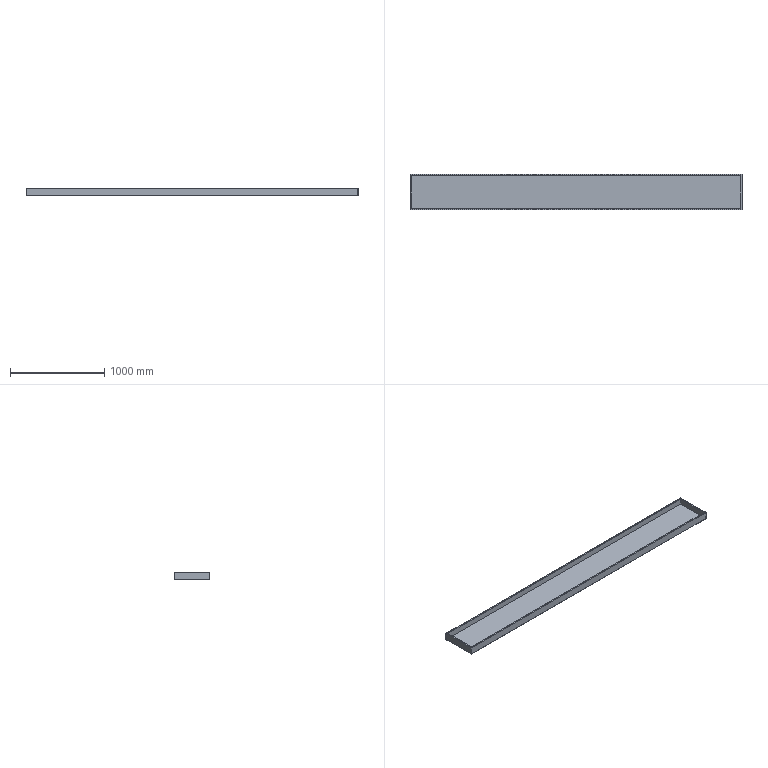Component | NX | DB3 | 1 solid | 16 faces | volume 3084987 mm3 | plane 16